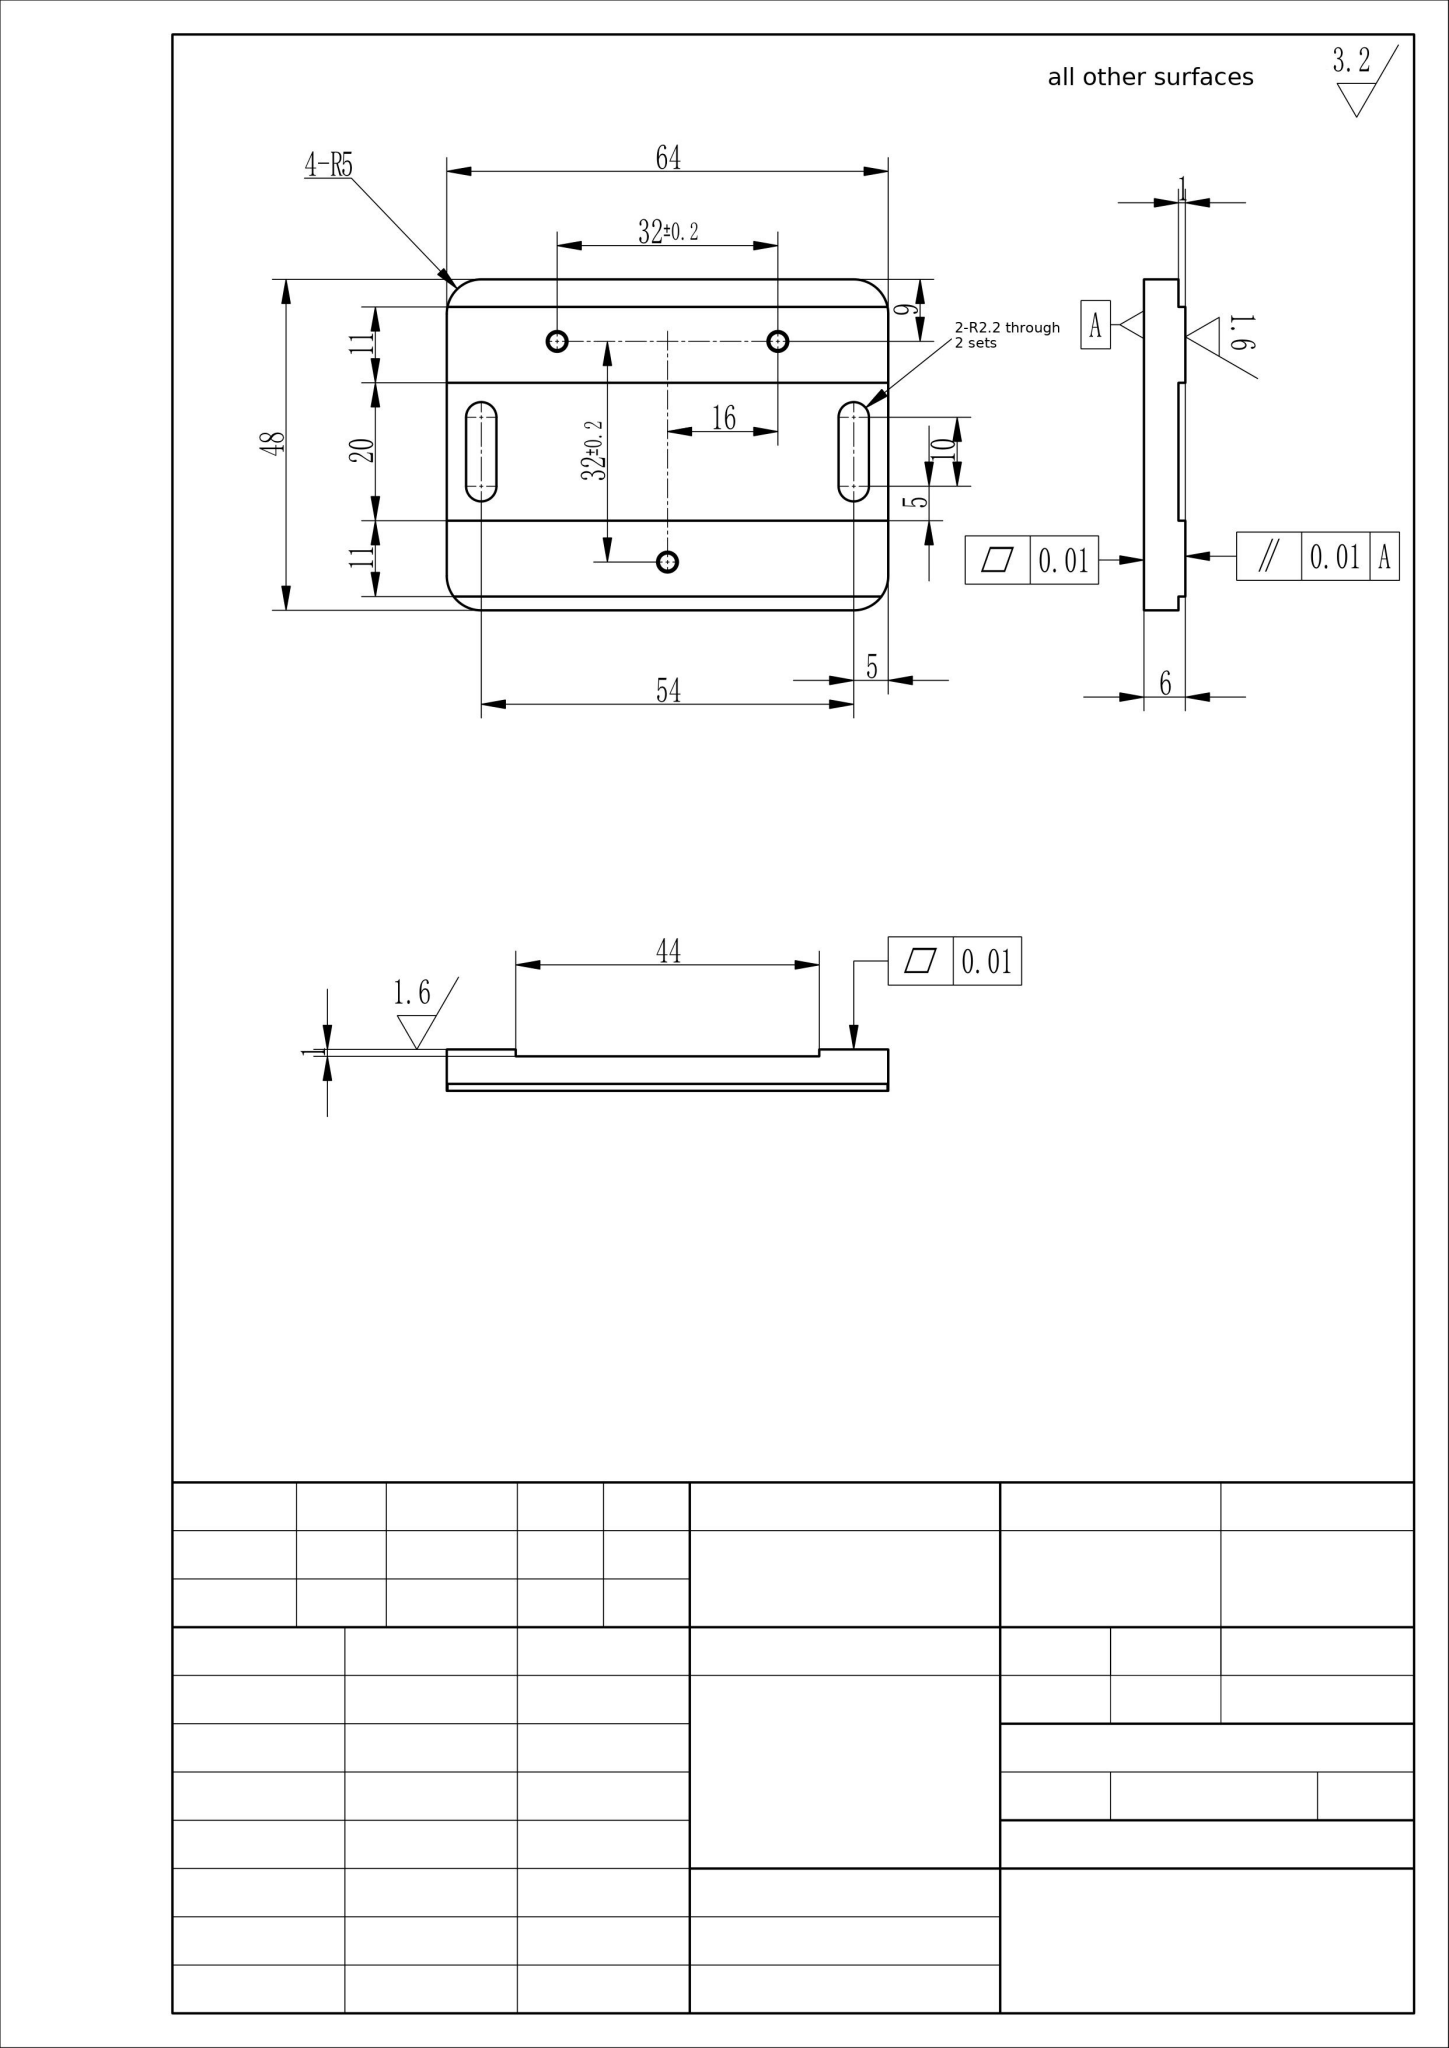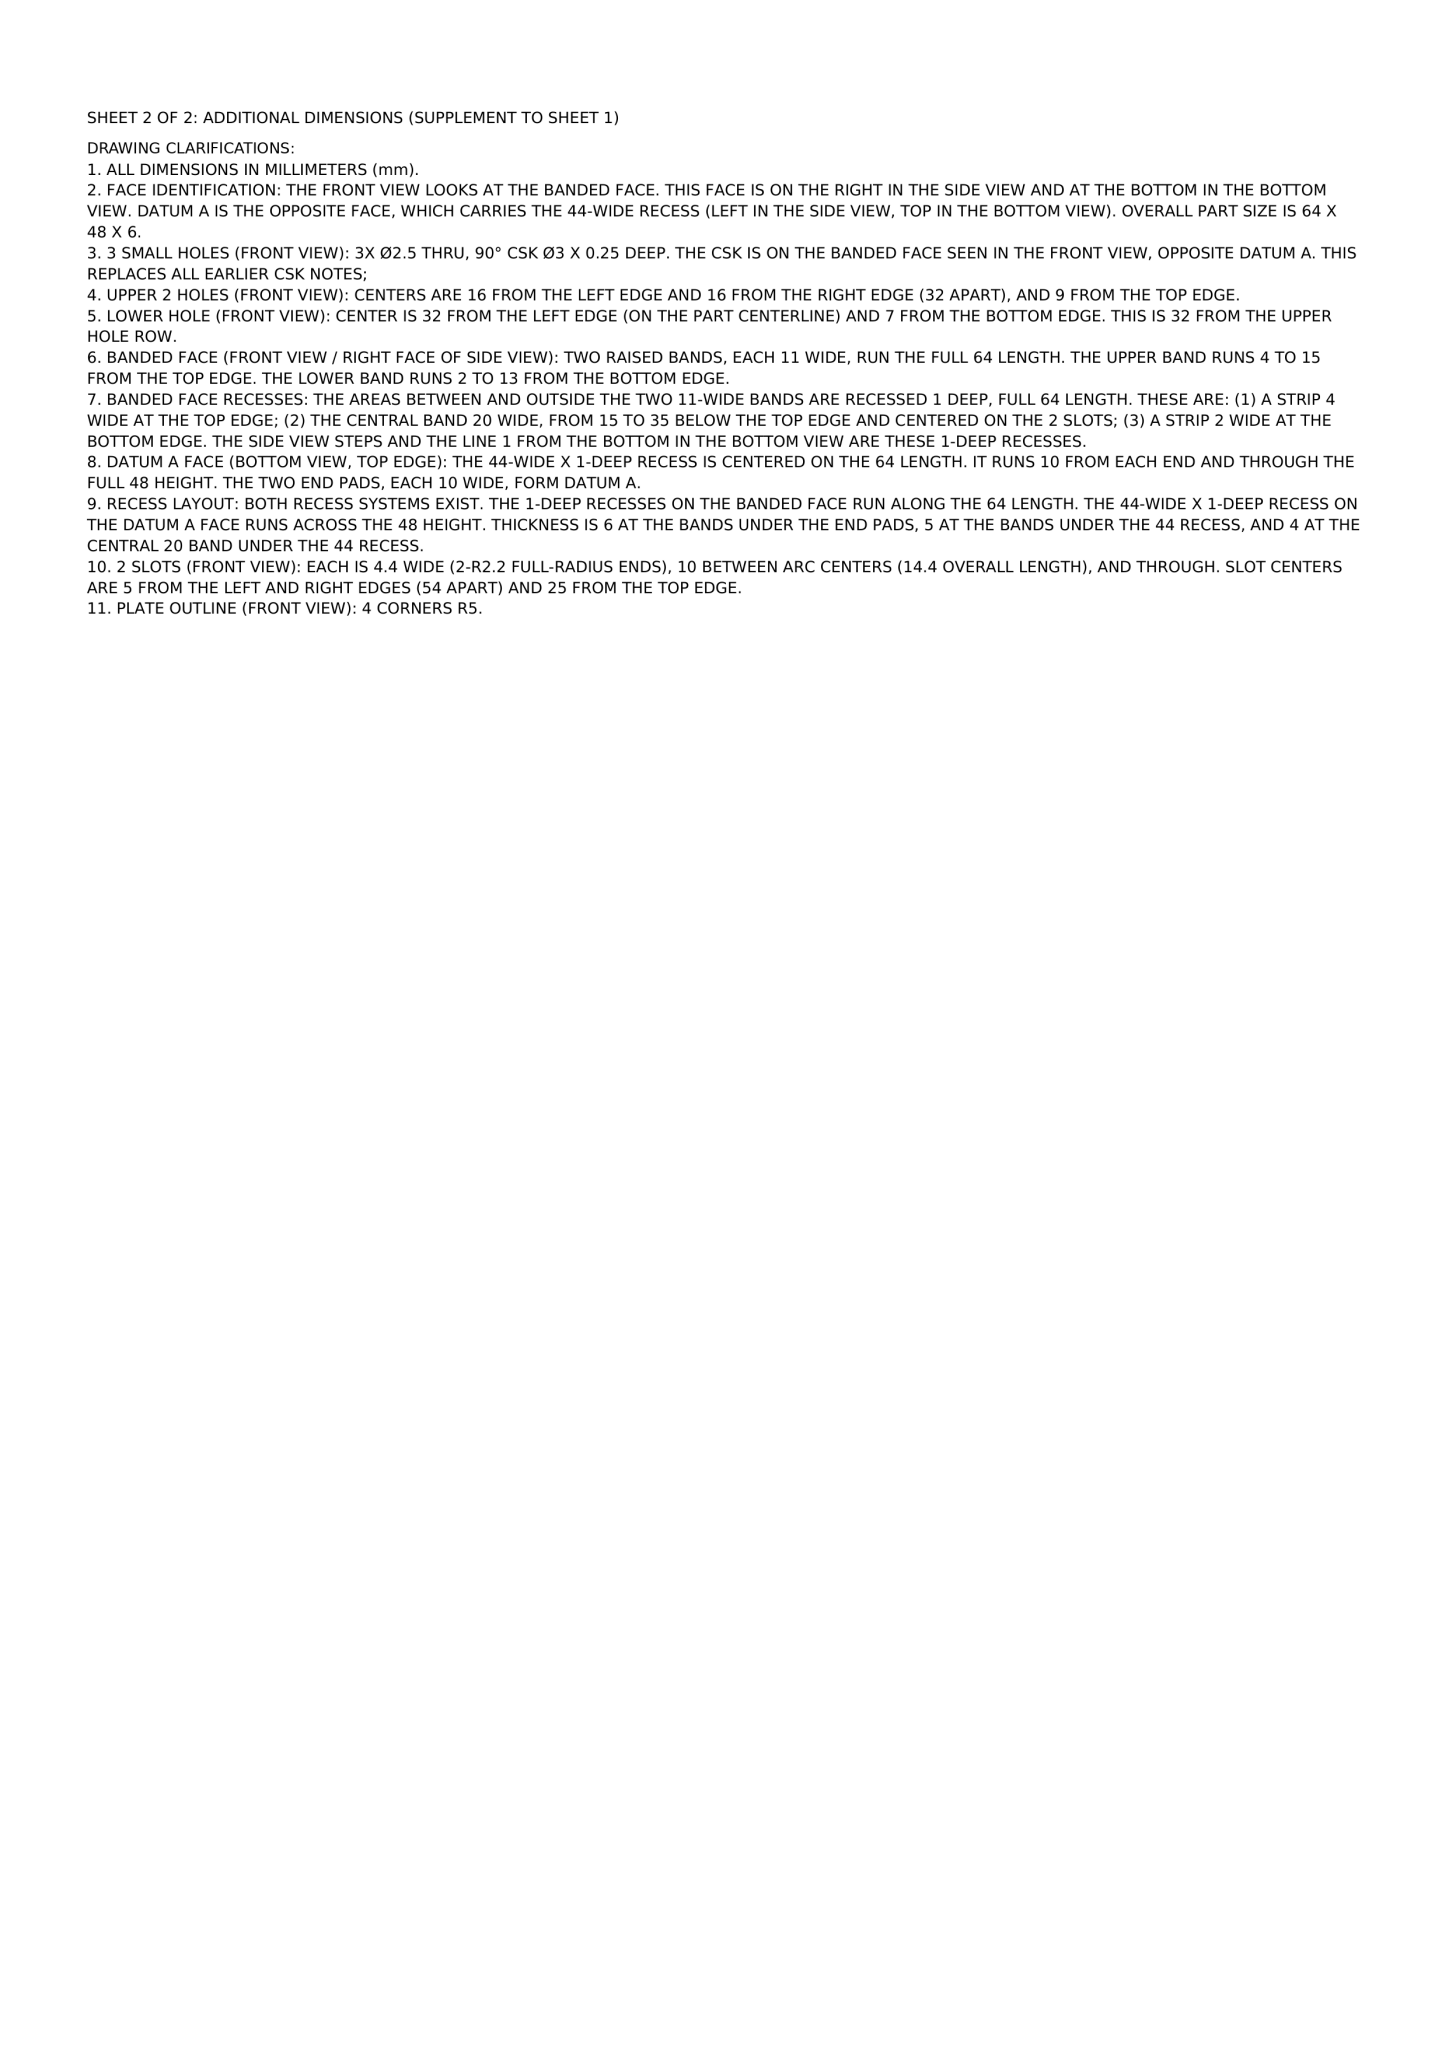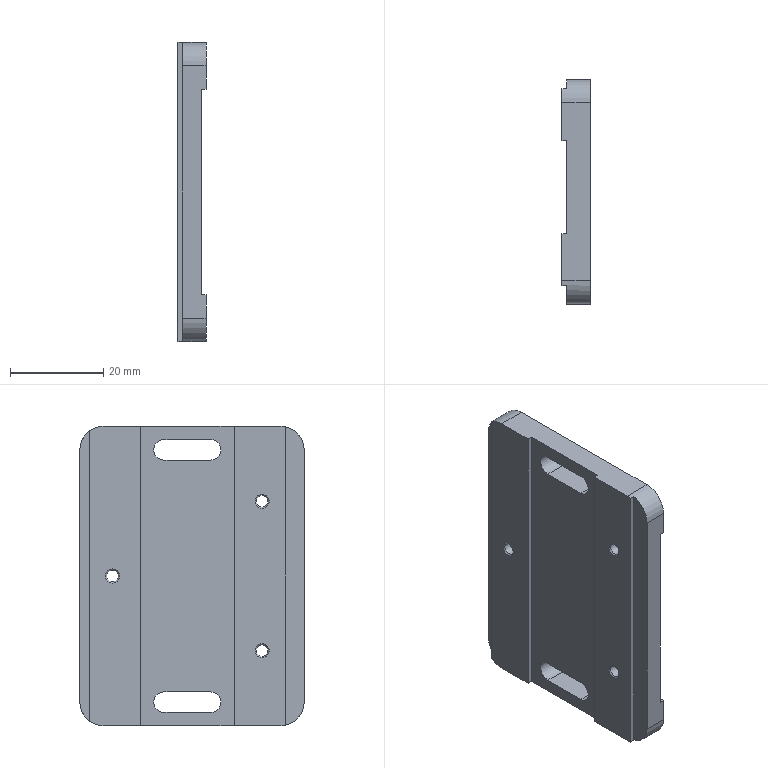Part | NX | mm | 1 solid | 36 faces | box 6 x 48 x 64 mm | volume 13880 mm3 | plane 22 | cylinder 11 | cone 3 | commonest cylinder face diameters 10 x4 4.4 x4 2.5 x3